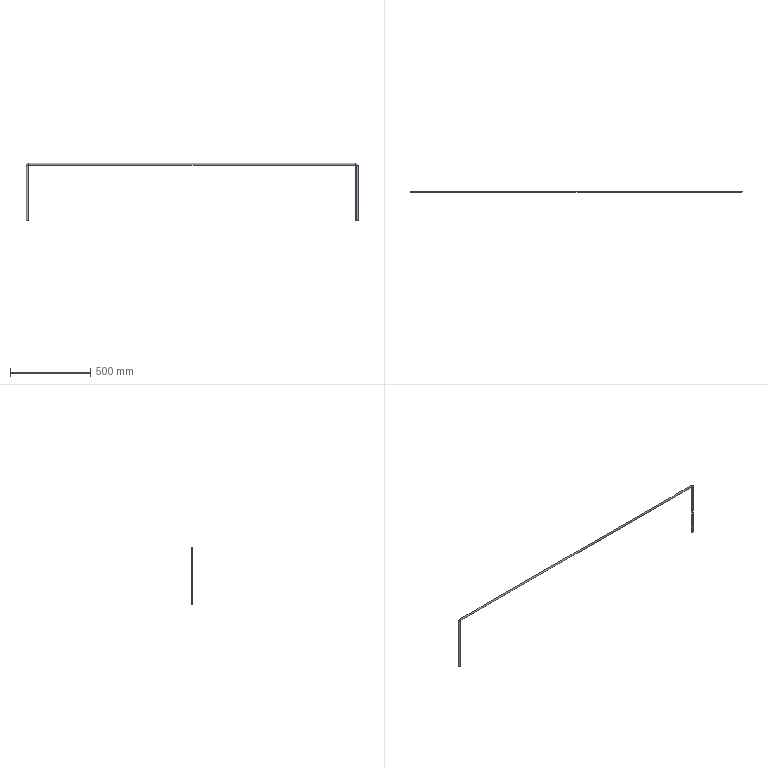Component | SolidWorks | LeftRearDoorAssembly-1_LeftRearDoorSealStrip-1 | 1 solid | 27 faces | volume 85065 mm3 | plane 21 | cylinder 4 | torus 2 | commonest cylinder face diameters 21.75 x4